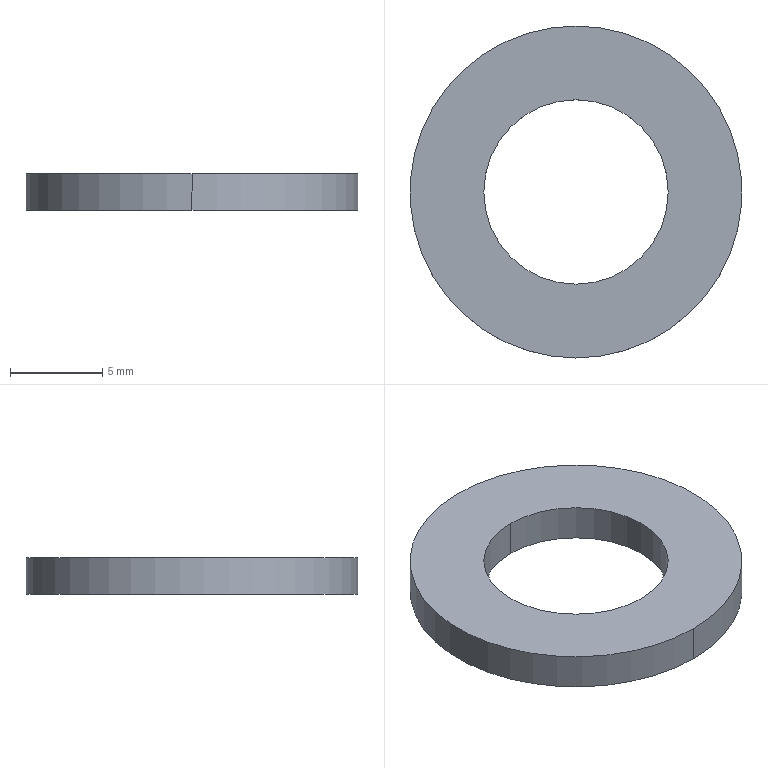Component | SolidWorks | ControlAssembly-1_UWAFN120-1_4_1-1 | 1 solid | 6 faces | box 18 x 18 x 2 mm | volume 352 mm3 | cylinder 4 | plane 2 | commonest cylinder face diameters 18 x2 10 x2
STEP:
#1=COLOUR_RGB('',0.7922,0.8196,0.9333);
#2=FILL_AREA_STYLE_COLOUR('',#1);
#3=FILL_AREA_STYLE('',(#2));
#4=SURFACE_STYLE_FILL_AREA(#3);
#5=SURFACE_SIDE_STYLE('',(#4));
#6=SURFACE_STYLE_USAGE(.BOTH.,#5);
#7=PRESENTATION_STYLE_ASSIGNMENT((#6));
#8=CARTESIAN_POINT('',(24.624,0.4554,20.569));
#9=VERTEX_POINT('',#8);
#10=CARTESIAN_POINT('',(24.624,1.164,20.569));
#11=VERTEX_POINT('',#10);
#12=CARTESIAN_POINT('',(24.624,0.8097,20.569));
#13=DIRECTION('',(-0.00009864,0.,-1.));
#14=DIRECTION('',(0.,1.,0.));
#15=AXIS2_PLACEMENT_3D('',#12,#13,#14);
#16=CIRCLE('',#15,0.3543);
#17=EDGE_CURVE('',#9,#11,#16,.T.);
#18=ORIENTED_EDGE('',*,*,#17,.F.);
#19=CARTESIAN_POINT('',(24.624,0.4554,20.648));
#20=VERTEX_POINT('',#19);
#21=CARTESIAN_POINT('',(24.624,0.4554,20.608));
#22=DIRECTION('',(0.00009864,-0.,1.));
#23=VECTOR('',#22,39.37);
#24=LINE('',#21,#23);
#25=EDGE_CURVE('',#9,#20,#24,.T.);
#26=ORIENTED_EDGE('',*,*,#25,.T.);
#27=CARTESIAN_POINT('',(24.624,1.164,20.648));
#28=VERTEX_POINT('',#27);
#29=CARTESIAN_POINT('',(24.624,0.8097,20.648));
#30=DIRECTION('',(-0.00009864,0.,-1.));
#31=DIRECTION('',(0.,1.,0.));
#32=AXIS2_PLACEMENT_3D('',#29,#30,#31);
#33=CIRCLE('',#32,0.3543);
#34=EDGE_CURVE('',#20,#28,#33,.T.);
#35=ORIENTED_EDGE('',*,*,#34,.T.);
#36=CARTESIAN_POINT('',(24.624,1.164,20.608));
#37=DIRECTION('',(0.00009864,-0.,1.));
#38=VECTOR('',#37,39.37);
#39=LINE('',#36,#38);
#40=EDGE_CURVE('',#11,#28,#39,.T.);
#41=ORIENTED_EDGE('',*,*,#40,.F.);
#42=EDGE_LOOP('',(#18,#26,#35,#41));
#43=FACE_OUTER_BOUND('',#42,.T.);
#44=CARTESIAN_POINT('',(24.624,0.8097,20.608));
#45=DIRECTION('',(0.00009864,-0.,1.));
#46=DIRECTION('',(0.,1.,0.));
#47=AXIS2_PLACEMENT_3D('',#44,#45,#46);
#48=CYLINDRICAL_SURFACE('',#47,0.3543);
#49=ADVANCED_FACE('',(#43),#48,.T.);
#50=CARTESIAN_POINT('',(24.624,0.6129,20.569));
#51=VERTEX_POINT('',#50);
#52=CARTESIAN_POINT('',(24.624,1.007,20.569));
#53=VERTEX_POINT('',#52);
#54=CARTESIAN_POINT('',(24.624,0.8097,20.569));
#55=DIRECTION('',(0.00009864,-0.,1.));
#56=DIRECTION('',(0.,1.,0.));
#57=AXIS2_PLACEMENT_3D('',#54,#55,#56);
#58=CIRCLE('',#57,0.1969);
#59=EDGE_CURVE('',#51,#53,#58,.T.);
#60=ORIENTED_EDGE('',*,*,#59,.F.);
#61=CARTESIAN_POINT('',(24.624,0.6129,20.648));
#62=VERTEX_POINT('',#61);
#63=CARTESIAN_POINT('',(24.624,0.6129,20.608));
#64=DIRECTION('',(0.00009864,-0.,1.));
#65=VECTOR('',#64,39.37);
#66=LINE('',#63,#65);
#67=EDGE_CURVE('',#51,#62,#66,.T.);
#68=ORIENTED_EDGE('',*,*,#67,.T.);
#69=CARTESIAN_POINT('',(24.624,1.007,20.648));
#70=VERTEX_POINT('',#69);
#71=CARTESIAN_POINT('',(24.624,0.8097,20.648));
#72=DIRECTION('',(-0.00009864,0.,-1.));
#73=DIRECTION('',(0.,1.,0.));
#74=AXIS2_PLACEMENT_3D('',#71,#72,#73);
#75=CIRCLE('',#74,0.1969);
#76=EDGE_CURVE('',#70,#62,#75,.T.);
#77=ORIENTED_EDGE('',*,*,#76,.F.);
#78=CARTESIAN_POINT('',(24.624,1.007,20.608));
#79=DIRECTION('',(0.00009864,-0.,1.));
#80=VECTOR('',#79,39.37);
#81=LINE('',#78,#80);
#82=EDGE_CURVE('',#53,#70,#81,.T.);
#83=ORIENTED_EDGE('',*,*,#82,.F.);
#84=EDGE_LOOP('',(#60,#68,#77,#83));
#85=FACE_OUTER_BOUND('',#84,.T.);
#86=CARTESIAN_POINT('',(24.624,0.8097,20.608));
#87=DIRECTION('',(0.00009864,-0.,1.));
#88=DIRECTION('',(0.,1.,0.));
#89=AXIS2_PLACEMENT_3D('',#86,#87,#88);
#90=CYLINDRICAL_SURFACE('',#89,0.1969);
#91=ADVANCED_FACE('',(#85),#90,.F.);
#92=CARTESIAN_POINT('',(24.624,0.8097,20.569));
#93=DIRECTION('',(-0.00009864,0.,-1.));
#94=DIRECTION('',(0.,1.,0.));
#95=AXIS2_PLACEMENT_3D('',#92,#93,#94);
#96=CIRCLE('',#95,0.3543);
#97=EDGE_CURVE('',#11,#9,#96,.T.);
#98=ORIENTED_EDGE('',*,*,#97,.T.);
#99=ORIENTED_EDGE('',*,*,#17,.T.);
#100=EDGE_LOOP('',(#98,#99));
#101=FACE_OUTER_BOUND('',#100,.T.);
#102=CARTESIAN_POINT('',(24.624,0.8097,20.569));
#103=DIRECTION('',(0.00009864,-0.,1.));
#104=DIRECTION('',(0.,1.,0.));
#105=AXIS2_PLACEMENT_3D('',#102,#103,#104);
#106=CIRCLE('',#105,0.1969);
#107=EDGE_CURVE('',#53,#51,#106,.T.);
#108=ORIENTED_EDGE('',*,*,#107,.T.);
#109=ORIENTED_EDGE('',*,*,#59,.T.);
#110=EDGE_LOOP('',(#108,#109));
#111=FACE_BOUND('',#110,.T.);
#112=CARTESIAN_POINT('',(24.624,0.5341,20.569));
#113=DIRECTION('',(-0.00009864,0.,-1.));
#114=DIRECTION('',(0.,-1.,-0.));
#115=AXIS2_PLACEMENT_3D('',#112,#113,#114);
#116=PLANE('',#115);
#117=ADVANCED_FACE('',(#101,#111),#116,.T.);
#118=ORIENTED_EDGE('',*,*,#25,.F.);
#119=ORIENTED_EDGE('',*,*,#97,.F.);
#120=ORIENTED_EDGE('',*,*,#40,.T.);
#121=CARTESIAN_POINT('',(24.624,0.8097,20.648));
#122=DIRECTION('',(-0.00009864,0.,-1.));
#123=DIRECTION('',(0.,1.,0.));
#124=AXIS2_PLACEMENT_3D('',#121,#122,#123);
#125=CIRCLE('',#124,0.3543);
#126=EDGE_CURVE('',#28,#20,#125,.T.);
#127=ORIENTED_EDGE('',*,*,#126,.T.);
#128=EDGE_LOOP('',(#118,#119,#120,#127));
#129=FACE_OUTER_BOUND('',#128,.T.);
#130=CARTESIAN_POINT('',(24.624,0.8097,20.608));
#131=DIRECTION('',(0.00009864,-0.,1.));
#132=DIRECTION('',(0.,1.,0.));
#133=AXIS2_PLACEMENT_3D('',#130,#131,#132);
#134=CYLINDRICAL_SURFACE('',#133,0.3543);
#135=ADVANCED_FACE('',(#129),#134,.T.);
#136=ORIENTED_EDGE('',*,*,#67,.F.);
#137=ORIENTED_EDGE('',*,*,#107,.F.);
#138=ORIENTED_EDGE('',*,*,#82,.T.);
#139=CARTESIAN_POINT('',(24.624,0.8097,20.648));
#140=DIRECTION('',(-0.00009864,0.,-1.));
#141=DIRECTION('',(0.,1.,0.));
#142=AXIS2_PLACEMENT_3D('',#139,#140,#141);
#143=CIRCLE('',#142,0.1969);
#144=EDGE_CURVE('',#62,#70,#143,.T.);
#145=ORIENTED_EDGE('',*,*,#144,.F.);
#146=EDGE_LOOP('',(#136,#137,#138,#145));
#147=FACE_OUTER_BOUND('',#146,.T.);
#148=CARTESIAN_POINT('',(24.624,0.8097,20.608));
#149=DIRECTION('',(0.00009864,-0.,1.));
#150=DIRECTION('',(0.,1.,0.));
#151=AXIS2_PLACEMENT_3D('',#148,#149,#150);
#152=CYLINDRICAL_SURFACE('',#151,0.1969);
#153=ADVANCED_FACE('',(#147),#152,.F.);
#154=ORIENTED_EDGE('',*,*,#76,.T.);
#155=ORIENTED_EDGE('',*,*,#144,.T.);
#156=EDGE_LOOP('',(#154,#155));
#157=FACE_BOUND('',#156,.T.);
#158=ORIENTED_EDGE('',*,*,#126,.F.);
#159=ORIENTED_EDGE('',*,*,#34,.F.);
#160=EDGE_LOOP('',(#158,#159));
#161=FACE_OUTER_BOUND('',#160,.T.);
#162=CARTESIAN_POINT('',(24.624,0.5341,20.648));
#163=DIRECTION('',(0.00009864,-0.,1.));
#164=DIRECTION('',(-0.,1.,0.));
#165=AXIS2_PLACEMENT_3D('',#162,#163,#164);
#166=PLANE('',#165);
#167=ADVANCED_FACE('',(#157,#161),#166,.T.);
#168=CLOSED_SHELL('',(#49,#91,#117,#135,#153,#167));
#169=MANIFOLD_SOLID_BREP('',#168);
#170=STYLED_ITEM('',(#7),#169);
#171=(LENGTH_UNIT()NAMED_UNIT(*)SI_UNIT($,.METRE.));
#172=LENGTH_MEASURE_WITH_UNIT(LENGTH_MEASURE(0.0254),#171);
#173=DIMENSIONAL_EXPONENTS(1.,0.,0.,0.,0.,0.,0.);
#174=(CONVERSION_BASED_UNIT('',#172)LENGTH_UNIT()NAMED_UNIT(#173));
#175=UNCERTAINTY_MEASURE_WITH_UNIT(LENGTH_MEASURE(0.00001),#174,'','');
#176=(NAMED_UNIT(*)PLANE_ANGLE_UNIT()SI_UNIT($,.RADIAN.));
#177=(NAMED_UNIT(*)SI_UNIT($,.STERADIAN.)SOLID_ANGLE_UNIT());
#178=(GEOMETRIC_REPRESENTATION_CONTEXT(3)GLOBAL_UNCERTAINTY_ASSIGNED_CONTEXT((#175))GLOBAL_UNIT_ASSIGNED_CONTEXT((#174,#176,#177))REPRESENTATION_CONTEXT('',''));
#179=MECHANICAL_DESIGN_GEOMETRIC_PRESENTATION_REPRESENTATION('',(#170),#178);
#180=CARTESIAN_POINT('',(0.,0.,0.));
#181=DIRECTION('',(0.,0.,1.));
#182=DIRECTION('',(1.,0.,0.));
#183=AXIS2_PLACEMENT_3D('',#180,#181,#182);
#184=(LENGTH_UNIT()NAMED_UNIT(*)SI_UNIT($,.METRE.));
#185=LENGTH_MEASURE_WITH_UNIT(LENGTH_MEASURE(0.0254),#184);
#186=DIMENSIONAL_EXPONENTS(1.,0.,0.,0.,0.,0.,0.);
#187=(CONVERSION_BASED_UNIT('',#185)LENGTH_UNIT()NAMED_UNIT(#186));
#188=UNCERTAINTY_MEASURE_WITH_UNIT(LENGTH_MEASURE(0.00001),#187,'','');
#189=(NAMED_UNIT(*)PLANE_ANGLE_UNIT()SI_UNIT($,.RADIAN.));
#190=(NAMED_UNIT(*)SI_UNIT($,.STERADIAN.)SOLID_ANGLE_UNIT());
#191=(GEOMETRIC_REPRESENTATION_CONTEXT(3)GLOBAL_UNCERTAINTY_ASSIGNED_CONTEXT((#188))GLOBAL_UNIT_ASSIGNED_CONTEXT((#187,#189,#190))REPRESENTATION_CONTEXT('',''));
#192=ADVANCED_BREP_SHAPE_REPRESENTATION('',(#169,#183),#191);
#193=PRESENTATION_LAYER_ASSIGNMENT('','',(#170));